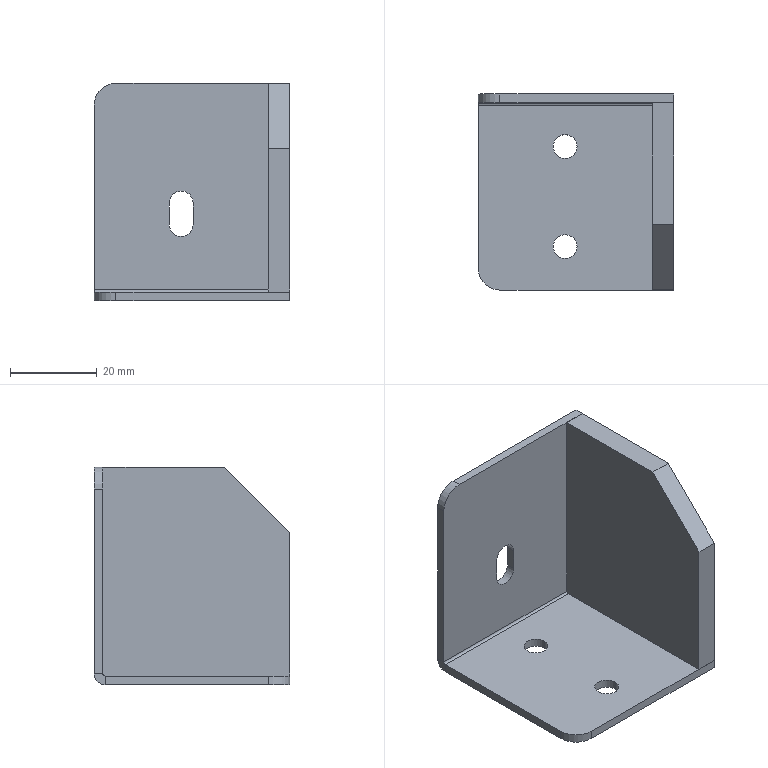Component | SolidWorks | 170423A4-ProfileSupportBlock-1 | 2 solids | 32 faces | box 45 x 45 x 50 mm | volume 17850 mm3 | plane 21 | cylinder 11 | commonest cylinder face diameters 5.5 x6 1 x2 10 x2 5 x1
STEP:
#1=COLOUR_RGB('',0.7922,0.8196,0.9333);
#2=FILL_AREA_STYLE_COLOUR('',#1);
#3=FILL_AREA_STYLE('',(#2));
#4=SURFACE_STYLE_FILL_AREA(#3);
#5=SURFACE_SIDE_STYLE('',(#4));
#6=SURFACE_STYLE_USAGE(.BOTH.,#5);
#7=PRESENTATION_STYLE_ASSIGNMENT((#6));
#8=CARTESIAN_POINT('',(3.248,-1.901,16.575));
#9=VERTEX_POINT('',#8);
#10=CARTESIAN_POINT('',(3.032,-1.901,16.575));
#11=VERTEX_POINT('',#10);
#12=CARTESIAN_POINT('',(3.14,-1.901,16.575));
#13=DIRECTION('',(0.,0.,1.));
#14=DIRECTION('',(-1.,0.,0.));
#15=AXIS2_PLACEMENT_3D('',#12,#13,#14);
#16=CIRCLE('',#15,0.1083);
#17=EDGE_CURVE('',#9,#11,#16,.T.);
#18=ORIENTED_EDGE('',*,*,#17,.F.);
#19=CARTESIAN_POINT('',(3.248,-1.901,16.654));
#20=VERTEX_POINT('',#19);
#21=CARTESIAN_POINT('',(3.248,-1.901,16.654));
#22=DIRECTION('',(0.,0.,1.));
#23=VECTOR('',#22,39.37);
#24=LINE('',#21,#23);
#25=EDGE_CURVE('',#9,#20,#24,.T.);
#26=ORIENTED_EDGE('',*,*,#25,.T.);
#27=CARTESIAN_POINT('',(3.032,-1.901,16.654));
#28=VERTEX_POINT('',#27);
#29=CARTESIAN_POINT('',(3.14,-1.901,16.654));
#30=DIRECTION('',(0.,0.,1.));
#31=DIRECTION('',(-1.,0.,0.));
#32=AXIS2_PLACEMENT_3D('',#29,#30,#31);
#33=CIRCLE('',#32,0.1083);
#34=EDGE_CURVE('',#20,#28,#33,.T.);
#35=ORIENTED_EDGE('',*,*,#34,.T.);
#36=CARTESIAN_POINT('',(3.032,-1.901,16.654));
#37=DIRECTION('',(0.,0.,1.));
#38=VECTOR('',#37,39.37);
#39=LINE('',#36,#38);
#40=EDGE_CURVE('',#11,#28,#39,.T.);
#41=ORIENTED_EDGE('',*,*,#40,.F.);
#42=EDGE_LOOP('',(#18,#26,#35,#41));
#43=FACE_OUTER_BOUND('',#42,.T.);
#44=CARTESIAN_POINT('',(3.14,-1.901,16.654));
#45=DIRECTION('',(0.,0.,1.));
#46=DIRECTION('',(-1.,0.,0.));
#47=AXIS2_PLACEMENT_3D('',#44,#45,#46);
#48=CYLINDRICAL_SURFACE('',#47,0.1083);
#49=ADVANCED_FACE('',(#43),#48,.F.);
#50=CARTESIAN_POINT('',(3.248,-2.807,16.575));
#51=VERTEX_POINT('',#50);
#52=CARTESIAN_POINT('',(3.032,-2.807,16.575));
#53=VERTEX_POINT('',#52);
#54=CARTESIAN_POINT('',(3.14,-2.807,16.575));
#55=DIRECTION('',(0.,0.,1.));
#56=DIRECTION('',(-1.,0.,0.));
#57=AXIS2_PLACEMENT_3D('',#54,#55,#56);
#58=CIRCLE('',#57,0.1083);
#59=EDGE_CURVE('',#51,#53,#58,.T.);
#60=ORIENTED_EDGE('',*,*,#59,.F.);
#61=CARTESIAN_POINT('',(3.248,-2.807,16.654));
#62=VERTEX_POINT('',#61);
#63=CARTESIAN_POINT('',(3.248,-2.807,16.654));
#64=DIRECTION('',(0.,0.,1.));
#65=VECTOR('',#64,39.37);
#66=LINE('',#63,#65);
#67=EDGE_CURVE('',#51,#62,#66,.T.);
#68=ORIENTED_EDGE('',*,*,#67,.T.);
#69=CARTESIAN_POINT('',(3.032,-2.807,16.654));
#70=VERTEX_POINT('',#69);
#71=CARTESIAN_POINT('',(3.14,-2.807,16.654));
#72=DIRECTION('',(0.,0.,1.));
#73=DIRECTION('',(-1.,0.,0.));
#74=AXIS2_PLACEMENT_3D('',#71,#72,#73);
#75=CIRCLE('',#74,0.1083);
#76=EDGE_CURVE('',#62,#70,#75,.T.);
#77=ORIENTED_EDGE('',*,*,#76,.T.);
#78=CARTESIAN_POINT('',(3.032,-2.807,16.654));
#79=DIRECTION('',(0.,0.,1.));
#80=VECTOR('',#79,39.37);
#81=LINE('',#78,#80);
#82=EDGE_CURVE('',#53,#70,#81,.T.);
#83=ORIENTED_EDGE('',*,*,#82,.F.);
#84=EDGE_LOOP('',(#60,#68,#77,#83));
#85=FACE_OUTER_BOUND('',#84,.T.);
#86=CARTESIAN_POINT('',(3.14,-2.807,16.654));
#87=DIRECTION('',(0.,0.,1.));
#88=DIRECTION('',(-1.,0.,0.));
#89=AXIS2_PLACEMENT_3D('',#86,#87,#88);
#90=CYLINDRICAL_SURFACE('',#89,0.1083);
#91=ADVANCED_FACE('',(#85),#90,.F.);
#92=CARTESIAN_POINT('',(2.353,-1.429,16.673));
#93=VERTEX_POINT('',#92);
#94=CARTESIAN_POINT('',(2.353,-1.507,16.673));
#95=VERTEX_POINT('',#94);
#96=CARTESIAN_POINT('',(2.353,-1.429,16.673));
#97=DIRECTION('',(0.,-1.,0.));
#98=VECTOR('',#97,39.37);
#99=LINE('',#96,#98);
#100=EDGE_CURVE('',#93,#95,#99,.T.);
#101=ORIENTED_EDGE('',*,*,#100,.F.);
#102=CARTESIAN_POINT('',(2.353,-1.527,16.575));
#103=VERTEX_POINT('',#102);
#104=CARTESIAN_POINT('',(2.353,-1.527,16.673));
#105=DIRECTION('',(-1.,-0.,0.));
#106=DIRECTION('',(0.,1.,0.));
#107=AXIS2_PLACEMENT_3D('',#104,#105,#106);
#108=CIRCLE('',#107,0.09843);
#109=EDGE_CURVE('',#93,#103,#108,.T.);
#110=ORIENTED_EDGE('',*,*,#109,.T.);
#111=CARTESIAN_POINT('',(2.353,-1.527,16.654));
#112=VERTEX_POINT('',#111);
#113=CARTESIAN_POINT('',(2.353,-1.527,16.654));
#114=DIRECTION('',(0.,0.,-1.));
#115=VECTOR('',#114,39.37);
#116=LINE('',#113,#115);
#117=EDGE_CURVE('',#112,#103,#116,.T.);
#118=ORIENTED_EDGE('',*,*,#117,.F.);
#119=CARTESIAN_POINT('',(2.353,-1.527,16.673));
#120=DIRECTION('',(-1.,-0.,0.));
#121=DIRECTION('',(0.,-1.,0.));
#122=AXIS2_PLACEMENT_3D('',#119,#120,#121);
#123=CIRCLE('',#122,0.01969);
#124=EDGE_CURVE('',#95,#112,#123,.T.);
#125=ORIENTED_EDGE('',*,*,#124,.F.);
#126=EDGE_LOOP('',(#101,#110,#118,#125));
#127=FACE_OUTER_BOUND('',#126,.T.);
#128=CARTESIAN_POINT('',(2.353,-1.429,16.673));
#129=DIRECTION('',(-1.,-0.,0.));
#130=DIRECTION('',(0.,-1.,0.));
#131=AXIS2_PLACEMENT_3D('',#128,#129,#130);
#132=PLANE('',#131);
#133=ADVANCED_FACE('',(#127),#132,.T.);
#134=CARTESIAN_POINT('',(2.353,-1.507,18.346));
#135=VERTEX_POINT('',#134);
#136=CARTESIAN_POINT('',(2.353,-1.507,16.575));
#137=DIRECTION('',(0.,0.,-1.));
#138=VECTOR('',#137,39.37);
#139=LINE('',#136,#138);
#140=EDGE_CURVE('',#135,#95,#139,.T.);
#141=ORIENTED_EDGE('',*,*,#140,.F.);
#142=CARTESIAN_POINT('',(2.353,-1.429,18.346));
#143=VERTEX_POINT('',#142);
#144=CARTESIAN_POINT('',(2.353,-1.527,18.346));
#145=DIRECTION('',(-0.,1.,0.));
#146=VECTOR('',#145,39.37);
#147=LINE('',#144,#146);
#148=EDGE_CURVE('',#135,#143,#147,.T.);
#149=ORIENTED_EDGE('',*,*,#148,.T.);
#150=CARTESIAN_POINT('',(2.353,-1.429,16.575));
#151=DIRECTION('',(0.,0.,-1.));
#152=VECTOR('',#151,39.37);
#153=LINE('',#150,#152);
#154=EDGE_CURVE('',#143,#93,#153,.T.);
#155=ORIENTED_EDGE('',*,*,#154,.T.);
#156=ORIENTED_EDGE('',*,*,#100,.T.);
#157=EDGE_LOOP('',(#141,#149,#155,#156));
#158=FACE_OUTER_BOUND('',#157,.T.);
#159=CARTESIAN_POINT('',(2.353,-1.527,16.654));
#160=DIRECTION('',(-1.,-0.,0.));
#161=DIRECTION('',(0.,-1.,0.));
#162=AXIS2_PLACEMENT_3D('',#159,#160,#161);
#163=PLANE('',#162);
#164=ADVANCED_FACE('',(#158),#163,.T.);
#165=CARTESIAN_POINT('',(4.124,-1.527,16.575));
#166=VERTEX_POINT('',#165);
#167=CARTESIAN_POINT('',(4.124,-1.527,16.654));
#168=VERTEX_POINT('',#167);
#169=CARTESIAN_POINT('',(4.124,-1.527,16.575));
#170=DIRECTION('',(0.,0.,1.));
#171=VECTOR('',#170,39.37);
#172=LINE('',#169,#171);
#173=EDGE_CURVE('',#166,#168,#172,.T.);
#174=ORIENTED_EDGE('',*,*,#173,.F.);
#175=CARTESIAN_POINT('',(4.124,-1.429,16.673));
#176=VERTEX_POINT('',#175);
#177=CARTESIAN_POINT('',(4.124,-1.527,16.673));
#178=DIRECTION('',(-1.,-0.,0.));
#179=DIRECTION('',(0.,1.,0.));
#180=AXIS2_PLACEMENT_3D('',#177,#178,#179);
#181=CIRCLE('',#180,0.09843);
#182=EDGE_CURVE('',#176,#166,#181,.T.);
#183=ORIENTED_EDGE('',*,*,#182,.F.);
#184=CARTESIAN_POINT('',(4.124,-1.507,16.673));
#185=VERTEX_POINT('',#184);
#186=CARTESIAN_POINT('',(4.124,-1.507,16.673));
#187=DIRECTION('',(-0.,1.,0.));
#188=VECTOR('',#187,39.37);
#189=LINE('',#186,#188);
#190=EDGE_CURVE('',#185,#176,#189,.T.);
#191=ORIENTED_EDGE('',*,*,#190,.F.);
#192=CARTESIAN_POINT('',(4.124,-1.527,16.673));
#193=DIRECTION('',(-1.,-0.,0.));
#194=DIRECTION('',(0.,-1.,0.));
#195=AXIS2_PLACEMENT_3D('',#192,#193,#194);
#196=CIRCLE('',#195,0.01969);
#197=EDGE_CURVE('',#185,#168,#196,.T.);
#198=ORIENTED_EDGE('',*,*,#197,.T.);
#199=EDGE_LOOP('',(#174,#183,#191,#198));
#200=FACE_OUTER_BOUND('',#199,.T.);
#201=CARTESIAN_POINT('',(4.124,-1.527,16.575));
#202=DIRECTION('',(1.,0.,0.));
#203=DIRECTION('',(-0.,1.,0.));
#204=AXIS2_PLACEMENT_3D('',#201,#202,#203);
#205=PLANE('',#204);
#206=ADVANCED_FACE('',(#200),#205,.T.);
#207=CARTESIAN_POINT('',(4.124,-3.2,16.575));
#208=VERTEX_POINT('',#207);
#209=CARTESIAN_POINT('',(4.124,-1.429,16.575));
#210=DIRECTION('',(0.,-1.,0.));
#211=VECTOR('',#210,39.37);
#212=LINE('',#209,#211);
#213=EDGE_CURVE('',#166,#208,#212,.T.);
#214=ORIENTED_EDGE('',*,*,#213,.F.);
#215=ORIENTED_EDGE('',*,*,#173,.T.);
#216=CARTESIAN_POINT('',(4.124,-3.2,16.654));
#217=VERTEX_POINT('',#216);
#218=CARTESIAN_POINT('',(4.124,-1.429,16.654));
#219=DIRECTION('',(0.,-1.,0.));
#220=VECTOR('',#219,39.37);
#221=LINE('',#218,#220);
#222=EDGE_CURVE('',#168,#217,#221,.T.);
#223=ORIENTED_EDGE('',*,*,#222,.T.);
#224=CARTESIAN_POINT('',(4.124,-3.2,16.654));
#225=DIRECTION('',(0.,0.,-1.));
#226=VECTOR('',#225,39.37);
#227=LINE('',#224,#226);
#228=EDGE_CURVE('',#217,#208,#227,.T.);
#229=ORIENTED_EDGE('',*,*,#228,.T.);
#230=EDGE_LOOP('',(#214,#215,#223,#229));
#231=FACE_OUTER_BOUND('',#230,.T.);
#232=CARTESIAN_POINT('',(4.124,-1.507,16.673));
#233=DIRECTION('',(1.,0.,0.));
#234=DIRECTION('',(-0.,1.,0.));
#235=AXIS2_PLACEMENT_3D('',#232,#233,#234);
#236=PLANE('',#235);
#237=ADVANCED_FACE('',(#231),#236,.T.);
#238=CARTESIAN_POINT('',(3.14,-1.901,16.575));
#239=DIRECTION('',(0.,0.,1.));
#240=DIRECTION('',(-1.,0.,0.));
#241=AXIS2_PLACEMENT_3D('',#238,#239,#240);
#242=CIRCLE('',#241,0.1083);
#243=EDGE_CURVE('',#11,#9,#242,.T.);
#244=ORIENTED_EDGE('',*,*,#243,.T.);
#245=ORIENTED_EDGE('',*,*,#17,.T.);
#246=EDGE_LOOP('',(#244,#245));
#247=FACE_BOUND('',#246,.T.);
#248=CARTESIAN_POINT('',(3.14,-2.807,16.575));
#249=DIRECTION('',(0.,0.,1.));
#250=DIRECTION('',(-1.,0.,0.));
#251=AXIS2_PLACEMENT_3D('',#248,#249,#250);
#252=CIRCLE('',#251,0.1083);
#253=EDGE_CURVE('',#53,#51,#252,.T.);
#254=ORIENTED_EDGE('',*,*,#253,.T.);
#255=ORIENTED_EDGE('',*,*,#59,.T.);
#256=EDGE_LOOP('',(#254,#255));
#257=FACE_BOUND('',#256,.T.);
#258=CARTESIAN_POINT('',(2.549,-3.2,16.575));
#259=VERTEX_POINT('',#258);
#260=CARTESIAN_POINT('',(2.353,-3.2,16.575));
#261=DIRECTION('',(1.,0.,0.));
#262=VECTOR('',#261,39.37);
#263=LINE('',#260,#262);
#264=EDGE_CURVE('',#259,#208,#263,.T.);
#265=ORIENTED_EDGE('',*,*,#264,.F.);
#266=CARTESIAN_POINT('',(2.353,-3.003,16.575));
#267=VERTEX_POINT('',#266);
#268=CARTESIAN_POINT('',(2.549,-3.003,16.575));
#269=DIRECTION('',(0.,0.,-1.));
#270=DIRECTION('',(-1.,-0.,0.));
#271=AXIS2_PLACEMENT_3D('',#268,#269,#270);
#272=CIRCLE('',#271,0.1969);
#273=EDGE_CURVE('',#259,#267,#272,.T.);
#274=ORIENTED_EDGE('',*,*,#273,.T.);
#275=CARTESIAN_POINT('',(2.353,-1.429,16.575));
#276=DIRECTION('',(0.,-1.,0.));
#277=VECTOR('',#276,39.37);
#278=LINE('',#275,#277);
#279=EDGE_CURVE('',#103,#267,#278,.T.);
#280=ORIENTED_EDGE('',*,*,#279,.F.);
#281=CARTESIAN_POINT('',(2.353,-1.527,16.575));
#282=DIRECTION('',(1.,0.,0.));
#283=VECTOR('',#282,39.37);
#284=LINE('',#281,#283);
#285=EDGE_CURVE('',#103,#166,#284,.T.);
#286=ORIENTED_EDGE('',*,*,#285,.T.);
#287=ORIENTED_EDGE('',*,*,#213,.T.);
#288=EDGE_LOOP('',(#265,#274,#280,#286,#287));
#289=FACE_OUTER_BOUND('',#288,.T.);
#290=CARTESIAN_POINT('',(2.353,-1.429,16.575));
#291=DIRECTION('',(0.,0.,1.));
#292=DIRECTION('',(-1.,-0.,0.));
#293=AXIS2_PLACEMENT_3D('',#290,#291,#292);
#294=PLANE('',#293);
#295=ADVANCED_FACE('',(#247,#257,#289),#294,.F.);
#296=CARTESIAN_POINT('',(2.549,-3.2,16.654));
#297=VERTEX_POINT('',#296);
#298=CARTESIAN_POINT('',(2.353,-3.2,16.654));
#299=DIRECTION('',(1.,0.,0.));
#300=VECTOR('',#299,39.37);
#301=LINE('',#298,#300);
#302=EDGE_CURVE('',#297,#217,#301,.T.);
#303=ORIENTED_EDGE('',*,*,#302,.F.);
#304=CARTESIAN_POINT('',(2.549,-3.2,16.654));
#305=DIRECTION('',(0.,0.,-1.));
#306=VECTOR('',#305,39.37);
#307=LINE('',#304,#306);
#308=EDGE_CURVE('',#297,#259,#307,.T.);
#309=ORIENTED_EDGE('',*,*,#308,.T.);
#310=ORIENTED_EDGE('',*,*,#264,.T.);
#311=ORIENTED_EDGE('',*,*,#228,.F.);
#312=EDGE_LOOP('',(#303,#309,#310,#311));
#313=FACE_OUTER_BOUND('',#312,.T.);
#314=CARTESIAN_POINT('',(2.353,-3.2,16.654));
#315=DIRECTION('',(0.,-1.,0.));
#316=DIRECTION('',(1.,0.,0.));
#317=AXIS2_PLACEMENT_3D('',#314,#315,#316);
#318=PLANE('',#317);
#319=ADVANCED_FACE('',(#313),#318,.T.);
#320=CARTESIAN_POINT('',(3.14,-1.901,16.654));
#321=DIRECTION('',(0.,0.,1.));
#322=DIRECTION('',(-1.,0.,0.));
#323=AXIS2_PLACEMENT_3D('',#320,#321,#322);
#324=CIRCLE('',#323,0.1083);
#325=EDGE_CURVE('',#28,#20,#324,.T.);
#326=ORIENTED_EDGE('',*,*,#325,.F.);
#327=ORIENTED_EDGE('',*,*,#34,.F.);
#328=EDGE_LOOP('',(#326,#327));
#329=FACE_BOUND('',#328,.T.);
#330=CARTESIAN_POINT('',(3.14,-2.807,16.654));
#331=DIRECTION('',(0.,0.,1.));
#332=DIRECTION('',(-1.,0.,0.));
#333=AXIS2_PLACEMENT_3D('',#330,#331,#332);
#334=CIRCLE('',#333,0.1083);
#335=EDGE_CURVE('',#70,#62,#334,.T.);
#336=ORIENTED_EDGE('',*,*,#335,.F.);
#337=ORIENTED_EDGE('',*,*,#76,.F.);
#338=EDGE_LOOP('',(#336,#337));
#339=FACE_BOUND('',#338,.T.);
#340=CARTESIAN_POINT('',(2.353,-3.003,16.654));
#341=VERTEX_POINT('',#340);
#342=CARTESIAN_POINT('',(2.353,-1.429,16.654));
#343=DIRECTION('',(0.,-1.,0.));
#344=VECTOR('',#343,39.37);
#345=LINE('',#342,#344);
#346=EDGE_CURVE('',#112,#341,#345,.T.);
#347=ORIENTED_EDGE('',*,*,#346,.T.);
#348=CARTESIAN_POINT('',(2.549,-3.003,16.654));
#349=DIRECTION('',(0.,0.,1.));
#350=DIRECTION('',(-1.,0.,0.));
#351=AXIS2_PLACEMENT_3D('',#348,#349,#350);
#352=CIRCLE('',#351,0.1969);
#353=EDGE_CURVE('',#341,#297,#352,.T.);
#354=ORIENTED_EDGE('',*,*,#353,.T.);
#355=ORIENTED_EDGE('',*,*,#302,.T.);
#356=ORIENTED_EDGE('',*,*,#222,.F.);
#357=CARTESIAN_POINT('',(2.353,-1.527,16.654));
#358=DIRECTION('',(1.,0.,0.));
#359=VECTOR('',#358,39.37);
#360=LINE('',#357,#359);
#361=EDGE_CURVE('',#112,#168,#360,.T.);
#362=ORIENTED_EDGE('',*,*,#361,.F.);
#363=EDGE_LOOP('',(#347,#354,#355,#356,#362));
#364=FACE_OUTER_BOUND('',#363,.T.);
#365=CARTESIAN_POINT('',(2.353,-1.429,16.654));
#366=DIRECTION('',(0.,0.,1.));
#367=DIRECTION('',(-1.,-0.,0.));
#368=AXIS2_PLACEMENT_3D('',#365,#366,#367);
#369=PLANE('',#368);
#370=ADVANCED_FACE('',(#329,#339,#364),#369,.T.);
#371=ORIENTED_EDGE('',*,*,#197,.F.);
#372=CARTESIAN_POINT('',(2.353,-1.507,16.673));
#373=DIRECTION('',(1.,0.,0.));
#374=VECTOR('',#373,39.37);
#375=LINE('',#372,#374);
#376=EDGE_CURVE('',#95,#185,#375,.T.);
#377=ORIENTED_EDGE('',*,*,#376,.F.);
#378=ORIENTED_EDGE('',*,*,#124,.T.);
#379=ORIENTED_EDGE('',*,*,#361,.T.);
#380=EDGE_LOOP('',(#371,#377,#378,#379));
#381=FACE_OUTER_BOUND('',#380,.T.);
#382=CARTESIAN_POINT('',(2.353,-1.527,16.673));
#383=DIRECTION('',(1.,0.,0.));
#384=DIRECTION('',(0.,1.,0.));
#385=AXIS2_PLACEMENT_3D('',#382,#383,#384);
#386=CYLINDRICAL_SURFACE('',#385,0.01969);
#387=ADVANCED_FACE('',(#381),#386,.F.);
#388=CARTESIAN_POINT('',(3.032,-1.507,17.264));
#389=VERTEX_POINT('',#388);
#390=CARTESIAN_POINT('',(3.248,-1.507,17.264));
#391=VERTEX_POINT('',#390);
#392=CARTESIAN_POINT('',(3.14,-1.507,17.264));
#393=DIRECTION('',(0.,-1.,0.));
#394=DIRECTION('',(1.,0.,0.));
#395=AXIS2_PLACEMENT_3D('',#392,#393,#394);
#396=CIRCLE('',#395,0.1083);
#397=EDGE_CURVE('',#389,#391,#396,.T.);
#398=ORIENTED_EDGE('',*,*,#397,.F.);
#399=CARTESIAN_POINT('',(3.032,-1.507,17.461));
#400=VERTEX_POINT('',#399);
#401=CARTESIAN_POINT('',(3.032,-1.507,17.264));
#402=DIRECTION('',(0.,0.,-1.));
#403=VECTOR('',#402,39.37);
#404=LINE('',#401,#403);
#405=EDGE_CURVE('',#400,#389,#404,.T.);
#406=ORIENTED_EDGE('',*,*,#405,.F.);
#407=CARTESIAN_POINT('',(3.248,-1.507,17.461));
#408=VERTEX_POINT('',#407);
#409=CARTESIAN_POINT('',(3.14,-1.507,17.461));
#410=DIRECTION('',(0.,-1.,0.));
#411=DIRECTION('',(1.,0.,0.));
#412=AXIS2_PLACEMENT_3D('',#409,#410,#411);
#413=CIRCLE('',#412,0.1083);
#414=EDGE_CURVE('',#408,#400,#413,.T.);
#415=ORIENTED_EDGE('',*,*,#414,.F.);
#416=CARTESIAN_POINT('',(3.248,-1.507,17.264));
#417=DIRECTION('',(0.,0.,1.));
#418=VECTOR('',#417,39.37);
#419=LINE('',#416,#418);
#420=EDGE_CURVE('',#391,#408,#419,.T.);
#421=ORIENTED_EDGE('',*,*,#420,.F.);
#422=EDGE_LOOP('',(#398,#406,#415,#421));
#423=FACE_BOUND('',#422,.T.);
#424=CARTESIAN_POINT('',(2.549,-1.507,18.543));
#425=VERTEX_POINT('',#424);
#426=CARTESIAN_POINT('',(4.124,-1.507,18.543));
#427=VERTEX_POINT('',#426);
#428=CARTESIAN_POINT('',(2.353,-1.507,18.543));
#429=DIRECTION('',(1.,0.,0.));
#430=VECTOR('',#429,39.37);
#431=LINE('',#428,#430);
#432=EDGE_CURVE('',#425,#427,#431,.T.);
#433=ORIENTED_EDGE('',*,*,#432,.F.);
#434=CARTESIAN_POINT('',(2.549,-1.507,18.346));
#435=DIRECTION('',(0.,-1.,0.));
#436=DIRECTION('',(1.,0.,0.));
#437=AXIS2_PLACEMENT_3D('',#434,#435,#436);
#438=CIRCLE('',#437,0.1969);
#439=EDGE_CURVE('',#425,#135,#438,.T.);
#440=ORIENTED_EDGE('',*,*,#439,.T.);
#441=ORIENTED_EDGE('',*,*,#140,.T.);
#442=ORIENTED_EDGE('',*,*,#376,.T.);
#443=CARTESIAN_POINT('',(4.124,-1.507,16.575));
#444=DIRECTION('',(0.,0.,-1.));
#445=VECTOR('',#444,39.37);
#446=LINE('',#443,#445);
#447=EDGE_CURVE('',#427,#185,#446,.T.);
#448=ORIENTED_EDGE('',*,*,#447,.F.);
#449=EDGE_LOOP('',(#433,#440,#441,#442,#448));
#450=FACE_OUTER_BOUND('',#449,.T.);
#451=CARTESIAN_POINT('',(2.353,-1.507,16.575));
#452=DIRECTION('',(0.,-1.,0.));
#453=DIRECTION('',(1.,0.,0.));
#454=AXIS2_PLACEMENT_3D('',#451,#452,#453);
#455=PLANE('',#454);
#456=ADVANCED_FACE('',(#423,#450),#455,.T.);
#457=CARTESIAN_POINT('',(2.549,-1.429,18.543));
#458=VERTEX_POINT('',#457);
#459=CARTESIAN_POINT('',(4.124,-1.429,18.543));
#460=VERTEX_POINT('',#459);
#461=CARTESIAN_POINT('',(2.353,-1.429,18.543));
#462=DIRECTION('',(1.,0.,0.));
#463=VECTOR('',#462,39.37);
#464=LINE('',#461,#463);
#465=EDGE_CURVE('',#458,#460,#464,.T.);
#466=ORIENTED_EDGE('',*,*,#465,.F.);
#467=CARTESIAN_POINT('',(2.549,-1.429,18.543));
#468=DIRECTION('',(0.,-1.,0.));
#469=VECTOR('',#468,39.37);
#470=LINE('',#467,#469);
#471=EDGE_CURVE('',#458,#425,#470,.T.);
#472=ORIENTED_EDGE('',*,*,#471,.T.);
#473=ORIENTED_EDGE('',*,*,#432,.T.);
#474=CARTESIAN_POINT('',(4.124,-1.429,18.543));
#475=DIRECTION('',(0.,-1.,0.));
#476=VECTOR('',#475,39.37);
#477=LINE('',#474,#476);
#478=EDGE_CURVE('',#460,#427,#477,.T.);
#479=ORIENTED_EDGE('',*,*,#478,.F.);
#480=EDGE_LOOP('',(#466,#472,#473,#479));
#481=FACE_OUTER_BOUND('',#480,.T.);
#482=CARTESIAN_POINT('',(2.353,-1.429,18.543));
#483=DIRECTION('',(0.,0.,1.));
#484=DIRECTION('',(-1.,-0.,0.));
#485=AXIS2_PLACEMENT_3D('',#482,#483,#484);
#486=PLANE('',#485);
#487=ADVANCED_FACE('',(#481),#486,.T.);
#488=CARTESIAN_POINT('',(3.032,-1.429,17.461));
#489=VERTEX_POINT('',#488);
#490=CARTESIAN_POINT('',(3.032,-1.429,17.264));
#491=VERTEX_POINT('',#490);
#492=CARTESIAN_POINT('',(3.032,-1.429,17.264));
#493=DIRECTION('',(0.,0.,-1.));
#494=VECTOR('',#493,39.37);
#495=LINE('',#492,#494);
#496=EDGE_CURVE('',#489,#491,#495,.T.);
#497=ORIENTED_EDGE('',*,*,#496,.T.);
#498=CARTESIAN_POINT('',(3.248,-1.429,17.264));
#499=VERTEX_POINT('',#498);
#500=CARTESIAN_POINT('',(3.14,-1.429,17.264));
#501=DIRECTION('',(0.,-1.,0.));
#502=DIRECTION('',(1.,0.,0.));
#503=AXIS2_PLACEMENT_3D('',#500,#501,#502);
#504=CIRCLE('',#503,0.1083);
#505=EDGE_CURVE('',#491,#499,#504,.T.);
#506=ORIENTED_EDGE('',*,*,#505,.T.);
#507=CARTESIAN_POINT('',(3.248,-1.429,17.461));
#508=VERTEX_POINT('',#507);
#509=CARTESIAN_POINT('',(3.248,-1.429,17.264));
#510=DIRECTION('',(0.,0.,1.));
#511=VECTOR('',#510,39.37);
#512=LINE('',#509,#511);
#513=EDGE_CURVE('',#499,#508,#512,.T.);
#514=ORIENTED_EDGE('',*,*,#513,.T.);
#515=CARTESIAN_POINT('',(3.14,-1.429,17.461));
#516=DIRECTION('',(0.,-1.,0.));
#517=DIRECTION('',(1.,0.,0.));
#518=AXIS2_PLACEMENT_3D('',#515,#516,#517);
#519=CIRCLE('',#518,0.1083);
#520=EDGE_CURVE('',#508,#489,#519,.T.);
#521=ORIENTED_EDGE('',*,*,#520,.T.);
#522=EDGE_LOOP('',(#497,#506,#514,#521));
#523=FACE_BOUND('',#522,.T.);
#524=ORIENTED_EDGE('',*,*,#154,.F.);
#525=CARTESIAN_POINT('',(2.549,-1.429,18.346));
#526=DIRECTION('',(-0.,1.,0.));
#527=DIRECTION('',(1.,0.,0.));
#528=AXIS2_PLACEMENT_3D('',#525,#526,#527);
#529=CIRCLE('',#528,0.1969);
#530=EDGE_CURVE('',#143,#458,#529,.T.);
#531=ORIENTED_EDGE('',*,*,#530,.T.);
#532=ORIENTED_EDGE('',*,*,#465,.T.);
#533=CARTESIAN_POINT('',(4.124,-1.429,16.575));
#534=DIRECTION('',(0.,0.,-1.));
#535=VECTOR('',#534,39.37);
#536=LINE('',#533,#535);
#537=EDGE_CURVE('',#460,#176,#536,.T.);
#538=ORIENTED_EDGE('',*,*,#537,.T.);
#539=CARTESIAN_POINT('',(2.353,-1.429,16.673));
#540=DIRECTION('',(1.,0.,0.));
#541=VECTOR('',#540,39.37);
#542=LINE('',#539,#541);
#543=EDGE_CURVE('',#93,#176,#542,.T.);
#544=ORIENTED_EDGE('',*,*,#543,.F.);
#545=EDGE_LOOP('',(#524,#531,#532,#538,#544));
#546=FACE_OUTER_BOUND('',#545,.T.);
#547=CARTESIAN_POINT('',(2.353,-1.429,16.575));
#548=DIRECTION('',(0.,-1.,0.));
#549=DIRECTION('',(1.,0.,0.));
#550=AXIS2_PLACEMENT_3D('',#547,#548,#549);
#551=PLANE('',#550);
#552=ADVANCED_FACE('',(#523,#546),#551,.F.);
#553=ORIENTED_EDGE('',*,*,#182,.T.);
#554=ORIENTED_EDGE('',*,*,#285,.F.);
#555=ORIENTED_EDGE('',*,*,#109,.F.);
#556=ORIENTED_EDGE('',*,*,#543,.T.);
#557=EDGE_LOOP('',(#553,#554,#555,#556));
#558=FACE_OUTER_BOUND('',#557,.T.);
#559=CARTESIAN_POINT('',(2.353,-1.527,16.673));
#560=DIRECTION('',(1.,0.,0.));
#561=DIRECTION('',(0.,1.,0.));
#562=AXIS2_PLACEMENT_3D('',#559,#560,#561);
#563=CYLINDRICAL_SURFACE('',#562,0.09843);
#564=ADVANCED_FACE('',(#558),#563,.T.);
#565=ORIENTED_EDGE('',*,*,#279,.T.);
#566=CARTESIAN_POINT('',(2.353,-3.003,16.673));
#567=DIRECTION('',(0.,0.,1.));
#568=VECTOR('',#567,39.37);
#569=LINE('',#566,#568);
#570=EDGE_CURVE('',#267,#341,#569,.T.);
#571=ORIENTED_EDGE('',*,*,#570,.T.);
#572=ORIENTED_EDGE('',*,*,#346,.F.);
#573=ORIENTED_EDGE('',*,*,#117,.T.);
#574=EDGE_LOOP('',(#565,#571,#572,#573));
#575=FACE_OUTER_BOUND('',#574,.T.);
#576=CARTESIAN_POINT('',(2.353,-1.527,16.673));
#577=DIRECTION('',(-1.,-0.,0.));
#578=DIRECTION('',(0.,-1.,0.));
#579=AXIS2_PLACEMENT_3D('',#576,#577,#578);
#580=PLANE('',#579);
#581=ADVANCED_FACE('',(#575),#580,.T.);
#582=ORIENTED_EDGE('',*,*,#447,.T.);
#583=ORIENTED_EDGE('',*,*,#190,.T.);
#584=ORIENTED_EDGE('',*,*,#537,.F.);
#585=ORIENTED_EDGE('',*,*,#478,.T.);
#586=EDGE_LOOP('',(#582,#583,#584,#585));
#587=FACE_OUTER_BOUND('',#586,.T.);
#588=CARTESIAN_POINT('',(4.124,-1.527,16.673));
#589=DIRECTION('',(-1.,-0.,0.));
#590=DIRECTION('',(0.,-1.,0.));
#591=AXIS2_PLACEMENT_3D('',#588,#589,#590);
#592=PLANE('',#591);
#593=ADVANCED_FACE('',(#587),#592,.F.);
#594=ORIENTED_EDGE('',*,*,#397,.T.);
#595=CARTESIAN_POINT('',(3.248,-1.429,17.264));
#596=DIRECTION('',(0.,-1.,0.));
#597=VECTOR('',#596,39.37);
#598=LINE('',#595,#597);
#599=EDGE_CURVE('',#499,#391,#598,.T.);
#600=ORIENTED_EDGE('',*,*,#599,.F.);
#601=ORIENTED_EDGE('',*,*,#505,.F.);
#602=CARTESIAN_POINT('',(3.032,-1.429,17.264));
#603=DIRECTION('',(0.,-1.,0.));
#604=VECTOR('',#603,39.37);
#605=LINE('',#602,#604);
#606=EDGE_CURVE('',#491,#389,#605,.T.);
#607=ORIENTED_EDGE('',*,*,#606,.T.);
#608=EDGE_LOOP('',(#594,#600,#601,#607));
#609=FACE_OUTER_BOUND('',#608,.T.);
#610=CARTESIAN_POINT('',(3.14,-1.429,17.264));
#611=DIRECTION('',(0.,-1.,0.));
#612=DIRECTION('',(1.,0.,0.));
#613=AXIS2_PLACEMENT_3D('',#610,#611,#612);
#614=CYLINDRICAL_SURFACE('',#613,0.1083);
#615=ADVANCED_FACE('',(#609),#614,.F.);
#616=ORIENTED_EDGE('',*,*,#405,.T.);
#617=ORIENTED_EDGE('',*,*,#606,.F.);
#618=ORIENTED_EDGE('',*,*,#496,.F.);
#619=CARTESIAN_POINT('',(3.032,-1.429,17.461));
#620=DIRECTION('',(0.,-1.,0.));
#621=VECTOR('',#620,39.37);
#622=LINE('',#619,#621);
#623=EDGE_CURVE('',#489,#400,#622,.T.);
#624=ORIENTED_EDGE('',*,*,#623,.T.);
#625=EDGE_LOOP('',(#616,#617,#618,#624));
#626=FACE_OUTER_BOUND('',#625,.T.);
#627=CARTESIAN_POINT('',(3.032,-1.429,17.264));
#628=DIRECTION('',(-1.,-0.,0.));
#629=DIRECTION('',(0.,-1.,0.));
#630=AXIS2_PLACEMENT_3D('',#627,#628,#629);
#631=PLANE('',#630);
#632=ADVANCED_FACE('',(#626),#631,.F.);
#633=ORIENTED_EDGE('',*,*,#414,.T.);
#634=ORIENTED_EDGE('',*,*,#623,.F.);
#635=ORIENTED_EDGE('',*,*,#520,.F.);
#636=CARTESIAN_POINT('',(3.248,-1.429,17.461));
#637=DIRECTION('',(0.,-1.,0.));
#638=VECTOR('',#637,39.37);
#639=LINE('',#636,#638);
#640=EDGE_CURVE('',#508,#408,#639,.T.);
#641=ORIENTED_EDGE('',*,*,#640,.T.);
#642=EDGE_LOOP('',(#633,#634,#635,#641));
#643=FACE_OUTER_BOUND('',#642,.T.);
#644=CARTESIAN_POINT('',(3.14,-1.429,17.461));
#645=DIRECTION('',(0.,-1.,0.));
#646=DIRECTION('',(1.,0.,0.));
#647=AXIS2_PLACEMENT_3D('',#644,#645,#646);
#648=CYLINDRICAL_SURFACE('',#647,0.1083);
#649=ADVANCED_FACE('',(#643),#648,.F.);
#650=ORIENTED_EDGE('',*,*,#420,.T.);
#651=ORIENTED_EDGE('',*,*,#640,.F.);
#652=ORIENTED_EDGE('',*,*,#513,.F.);
#653=ORIENTED_EDGE('',*,*,#599,.T.);
#654=EDGE_LOOP('',(#650,#651,#652,#653));
#655=FACE_OUTER_BOUND('',#654,.T.);
#656=CARTESIAN_POINT('',(3.248,-1.429,17.264));
#657=DIRECTION('',(1.,0.,0.));
#658=DIRECTION('',(-0.,1.,0.));
#659=AXIS2_PLACEMENT_3D('',#656,#657,#658);
#660=PLANE('',#659);
#661=ADVANCED_FACE('',(#655),#660,.F.);
#662=ORIENTED_EDGE('',*,*,#353,.F.);
#663=ORIENTED_EDGE('',*,*,#570,.F.);
#664=ORIENTED_EDGE('',*,*,#273,.F.);
#665=ORIENTED_EDGE('',*,*,#308,.F.);
#666=EDGE_LOOP('',(#662,#663,#664,#665));
#667=FACE_OUTER_BOUND('',#666,.T.);
#668=CARTESIAN_POINT('',(2.549,-3.003,16.654));
#669=DIRECTION('',(0.,0.,-1.));
#670=DIRECTION('',(1.,0.,0.));
#671=AXIS2_PLACEMENT_3D('',#668,#669,#670);
#672=CYLINDRICAL_SURFACE('',#671,0.1969);
#673=ADVANCED_FACE('',(#667),#672,.T.);
#674=ORIENTED_EDGE('',*,*,#530,.F.);
#675=ORIENTED_EDGE('',*,*,#148,.F.);
#676=ORIENTED_EDGE('',*,*,#439,.F.);
#677=ORIENTED_EDGE('',*,*,#471,.F.);
#678=EDGE_LOOP('',(#674,#675,#676,#677));
#679=FACE_OUTER_BOUND('',#678,.T.);
#680=CARTESIAN_POINT('',(2.549,-1.429,18.346));
#681=DIRECTION('',(0.,-1.,0.));
#682=DIRECTION('',(1.,0.,0.));
#683=AXIS2_PLACEMENT_3D('',#680,#681,#682);
#684=CYLINDRICAL_SURFACE('',#683,0.1969);
#685=ADVANCED_FACE('',(#679),#684,.T.);
#686=ORIENTED_EDGE('',*,*,#67,.F.);
#687=ORIENTED_EDGE('',*,*,#253,.F.);
#688=ORIENTED_EDGE('',*,*,#82,.T.);
#689=ORIENTED_EDGE('',*,*,#335,.T.);
#690=EDGE_LOOP('',(#686,#687,#688,#689));
#691=FACE_OUTER_BOUND('',#690,.T.);
#692=CARTESIAN_POINT('',(3.14,-2.807,16.654));
#693=DIRECTION('',(0.,0.,1.));
#694=DIRECTION('',(-1.,0.,0.));
#695=AXIS2_PLACEMENT_3D('',#692,#693,#694);
#696=CYLINDRICAL_SURFACE('',#695,0.1083);
#697=ADVANCED_FACE('',(#691),#696,.F.);
#698=ORIENTED_EDGE('',*,*,#25,.F.);
#699=ORIENTED_EDGE('',*,*,#243,.F.);
#700=ORIENTED_EDGE('',*,*,#40,.T.);
#701=ORIENTED_EDGE('',*,*,#325,.T.);
#702=EDGE_LOOP('',(#698,#699,#700,#701));
#703=FACE_OUTER_BOUND('',#702,.T.);
#704=CARTESIAN_POINT('',(3.14,-1.901,16.654));
#705=DIRECTION('',(0.,0.,1.));
#706=DIRECTION('',(-1.,0.,0.));
#707=AXIS2_PLACEMENT_3D('',#704,#705,#706);
#708=CYLINDRICAL_SURFACE('',#707,0.1083);
#709=ADVANCED_FACE('',(#703),#708,.F.);
#710=CLOSED_SHELL('',(#49,#91,#133,#164,#206,#237,#295,#319,#370,#387,#456,#487,#552,#564,#581,#593,#615,#632,#649,#661,#673,#685,#697,#709));
#711=MANIFOLD_SOLID_BREP('',#710);
#712=STYLED_ITEM('',(#7),#711);
#713=(LENGTH_UNIT()NAMED_UNIT(*)SI_UNIT($,.METRE.));
#714=LENGTH_MEASURE_WITH_UNIT(LENGTH_MEASURE(0.0254),#713);
#715=DIMENSIONAL_EXPONENTS(1.,0.,0.,0.,0.,0.,0.);
#716=(CONVERSION_BASED_UNIT('',#714)LENGTH_UNIT()NAMED_UNIT(#715));
#717=UNCERTAINTY_MEASURE_WITH_UNIT(LENGTH_MEASURE(0.00001),#716,'','');
#718=(NAMED_UNIT(*)PLANE_ANGLE_UNIT()SI_UNIT($,.RADIAN.));
#719=(NAMED_UNIT(*)SI_UNIT($,.STERADIAN.)SOLID_ANGLE_UNIT());
#720=(GEOMETRIC_REPRESENTATION_CONTEXT(3)GLOBAL_UNCERTAINTY_ASSIGNED_CONTEXT((#717))GLOBAL_UNIT_ASSIGNED_CONTEXT((#716,#718,#719))REPRESENTATION_CONTEXT('',''));
#721=MECHANICAL_DESIGN_GEOMETRIC_PRESENTATION_REPRESENTATION('',(#712),#720);
#722=COLOUR_RGB('',0.7922,0.8196,0.9333);
#723=FILL_AREA_STYLE_COLOUR('',#722);
#724=FILL_AREA_STYLE('',(#723));
#725=SURFACE_STYLE_FILL_AREA(#724);
#726=SURFACE_SIDE_STYLE('',(#725));
#727=SURFACE_STYLE_USAGE(.BOTH.,#726);
#728=PRESENTATION_STYLE_ASSIGNMENT((#727));
#729=CARTESIAN_POINT('',(4.124,-1.527,16.654));
#730=VERTEX_POINT('',#729);
#731=CARTESIAN_POINT('',(4.124,-1.507,16.673));
#732=VERTEX_POINT('',#731);
#733=CARTESIAN_POINT('',(4.124,-1.527,16.673));
#734=DIRECTION('',(1.,0.,0.));
#735=DIRECTION('',(0.,1.,0.));
#736=AXIS2_PLACEMENT_3D('',#733,#734,#735);
#737=CIRCLE('',#736,0.01969);
#738=EDGE_CURVE('',#730,#732,#737,.T.);
#739=ORIENTED_EDGE('',*,*,#738,.F.);
#740=CARTESIAN_POINT('',(3.927,-1.527,16.654));
#741=VERTEX_POINT('',#740);
#742=CARTESIAN_POINT('',(3.927,-1.527,16.654));
#743=DIRECTION('',(1.,0.,0.));
#744=VECTOR('',#743,39.37);
#745=LINE('',#742,#744);
#746=EDGE_CURVE('',#741,#730,#745,.T.);
#747=ORIENTED_EDGE('',*,*,#746,.F.);
#748=CARTESIAN_POINT('',(3.927,-1.507,16.673));
#749=VERTEX_POINT('',#748);
#750=CARTESIAN_POINT('',(3.927,-1.527,16.673));
#751=DIRECTION('',(1.,0.,0.));
#752=DIRECTION('',(0.,1.,0.));
#753=AXIS2_PLACEMENT_3D('',#750,#751,#752);
#754=CIRCLE('',#753,0.01969);
#755=EDGE_CURVE('',#741,#749,#754,.T.);
#756=ORIENTED_EDGE('',*,*,#755,.T.);
#757=CARTESIAN_POINT('',(3.927,-1.507,16.673));
#758=DIRECTION('',(1.,0.,0.));
#759=VECTOR('',#758,39.37);
#760=LINE('',#757,#759);
#761=EDGE_CURVE('',#749,#732,#760,.T.);
#762=ORIENTED_EDGE('',*,*,#761,.T.);
#763=EDGE_LOOP('',(#739,#747,#756,#762));
#764=FACE_OUTER_BOUND('',#763,.T.);
#765=CARTESIAN_POINT('',(3.927,-1.527,16.673));
#766=DIRECTION('',(1.,0.,0.));
#767=DIRECTION('',(0.,1.,0.));
#768=AXIS2_PLACEMENT_3D('',#765,#766,#767);
#769=CYLINDRICAL_SURFACE('',#768,0.01969);
#770=ADVANCED_FACE('',(#764),#769,.T.);
#771=CARTESIAN_POINT('',(4.124,-3.2,16.654));
#772=VERTEX_POINT('',#771);
#773=CARTESIAN_POINT('',(4.124,-1.527,16.654));
#774=DIRECTION('',(-0.,1.,0.));
#775=VECTOR('',#774,39.37);
#776=LINE('',#773,#775);
#777=EDGE_CURVE('',#772,#730,#776,.T.);
#778=ORIENTED_EDGE('',*,*,#777,.F.);
#779=CARTESIAN_POINT('',(3.927,-3.2,16.654));
#780=VERTEX_POINT('',#779);
#781=CARTESIAN_POINT('',(3.927,-3.2,16.654));
#782=DIRECTION('',(1.,0.,0.));
#783=VECTOR('',#782,39.37);
#784=LINE('',#781,#783);
#785=EDGE_CURVE('',#780,#772,#784,.T.);
#786=ORIENTED_EDGE('',*,*,#785,.F.);
#787=CARTESIAN_POINT('',(3.927,-1.527,16.654));
#788=DIRECTION('',(-0.,1.,0.));
#789=VECTOR('',#788,39.37);
#790=LINE('',#787,#789);
#791=EDGE_CURVE('',#780,#741,#790,.T.);
#792=ORIENTED_EDGE('',*,*,#791,.T.);
#793=ORIENTED_EDGE('',*,*,#746,.T.);
#794=EDGE_LOOP('',(#778,#786,#792,#793));
#795=FACE_OUTER_BOUND('',#794,.T.);
#796=CARTESIAN_POINT('',(3.927,-1.527,16.654));
#797=DIRECTION('',(0.,0.,-1.));
#798=DIRECTION('',(1.,0.,0.));
#799=AXIS2_PLACEMENT_3D('',#796,#797,#798);
#800=PLANE('',#799);
#801=ADVANCED_FACE('',(#795),#800,.T.);
#802=CARTESIAN_POINT('',(4.124,-3.2,17.953));
#803=VERTEX_POINT('',#802);
#804=CARTESIAN_POINT('',(4.124,-3.2,18.543));
#805=DIRECTION('',(-0.,0.,-1.));
#806=VECTOR('',#805,39.37);
#807=LINE('',#804,#806);
#808=EDGE_CURVE('',#803,#772,#807,.T.);
#809=ORIENTED_EDGE('',*,*,#808,.F.);
#810=CARTESIAN_POINT('',(3.927,-3.2,17.953));
#811=VERTEX_POINT('',#810);
#812=CARTESIAN_POINT('',(3.927,-3.2,17.953));
#813=DIRECTION('',(-1.,-0.,0.));
#814=VECTOR('',#813,39.37);
#815=LINE('',#812,#814);
#816=EDGE_CURVE('',#803,#811,#815,.T.);
#817=ORIENTED_EDGE('',*,*,#816,.T.);
#818=CARTESIAN_POINT('',(3.927,-3.2,18.543));
#819=DIRECTION('',(-0.,0.,-1.));
#820=VECTOR('',#819,39.37);
#821=LINE('',#818,#820);
#822=EDGE_CURVE('',#811,#780,#821,.T.);
#823=ORIENTED_EDGE('',*,*,#822,.T.);
#824=ORIENTED_EDGE('',*,*,#785,.T.);
#825=EDGE_LOOP('',(#809,#817,#823,#824));
#826=FACE_OUTER_BOUND('',#825,.T.);
#827=CARTESIAN_POINT('',(3.927,-3.2,18.543));
#828=DIRECTION('',(0.,-1.,-0.));
#829=DIRECTION('',(0.,-0.,1.));
#830=AXIS2_PLACEMENT_3D('',#827,#828,#829);
#831=PLANE('',#830);
#832=ADVANCED_FACE('',(#826),#831,.T.);
#833=CARTESIAN_POINT('',(3.927,-1.507,18.543));
#834=VERTEX_POINT('',#833);
#835=CARTESIAN_POINT('',(3.927,-2.61,18.543));
#836=VERTEX_POINT('',#835);
#837=CARTESIAN_POINT('',(3.927,-1.507,18.543));
#838=DIRECTION('',(0.,-1.,-0.));
#839=VECTOR('',#838,39.37);
#840=LINE('',#837,#839);
#841=EDGE_CURVE('',#834,#836,#840,.T.);
#842=ORIENTED_EDGE('',*,*,#841,.T.);
#843=CARTESIAN_POINT('',(4.124,-2.61,18.543));
#844=VERTEX_POINT('',#843);
#845=CARTESIAN_POINT('',(3.927,-2.61,18.543));
#846=DIRECTION('',(1.,0.,0.));
#847=VECTOR('',#846,39.37);
#848=LINE('',#845,#847);
#849=EDGE_CURVE('',#836,#844,#848,.T.);
#850=ORIENTED_EDGE('',*,*,#849,.T.);
#851=CARTESIAN_POINT('',(4.124,-1.507,18.543));
#852=VERTEX_POINT('',#851);
#853=CARTESIAN_POINT('',(4.124,-1.507,18.543));
#854=DIRECTION('',(0.,-1.,-0.));
#855=VECTOR('',#854,39.37);
#856=LINE('',#853,#855);
#857=EDGE_CURVE('',#852,#844,#856,.T.);
#858=ORIENTED_EDGE('',*,*,#857,.F.);
#859=CARTESIAN_POINT('',(3.927,-1.507,18.543));
#860=DIRECTION('',(1.,0.,0.));
#861=VECTOR('',#860,39.37);
#862=LINE('',#859,#861);
#863=EDGE_CURVE('',#834,#852,#862,.T.);
#864=ORIENTED_EDGE('',*,*,#863,.F.);
#865=EDGE_LOOP('',(#842,#850,#858,#864));
#866=FACE_OUTER_BOUND('',#865,.T.);
#867=CARTESIAN_POINT('',(3.927,-1.507,18.543));
#868=DIRECTION('',(0.,-0.,1.));
#869=DIRECTION('',(-0.,1.,0.));
#870=AXIS2_PLACEMENT_3D('',#867,#868,#869);
#871=PLANE('',#870);
#872=ADVANCED_FACE('',(#866),#871,.T.);
#873=CARTESIAN_POINT('',(4.124,-1.507,18.543));
#874=DIRECTION('',(0.,0.,1.));
#875=VECTOR('',#874,39.37);
#876=LINE('',#873,#875);
#877=EDGE_CURVE('',#732,#852,#876,.T.);
#878=ORIENTED_EDGE('',*,*,#877,.F.);
#879=ORIENTED_EDGE('',*,*,#761,.F.);
#880=CARTESIAN_POINT('',(3.927,-1.507,18.543));
#881=DIRECTION('',(0.,0.,1.));
#882=VECTOR('',#881,39.37);
#883=LINE('',#880,#882);
#884=EDGE_CURVE('',#749,#834,#883,.T.);
#885=ORIENTED_EDGE('',*,*,#884,.T.);
#886=ORIENTED_EDGE('',*,*,#863,.T.);
#887=EDGE_LOOP('',(#878,#879,#885,#886));
#888=FACE_OUTER_BOUND('',#887,.T.);
#889=CARTESIAN_POINT('',(3.927,-1.507,18.543));
#890=DIRECTION('',(-0.,1.,0.));
#891=DIRECTION('',(-1.,-0.,0.));
#892=AXIS2_PLACEMENT_3D('',#889,#890,#891);
#893=PLANE('',#892);
#894=ADVANCED_FACE('',(#888),#893,.T.);
#895=ORIENTED_EDGE('',*,*,#822,.F.);
#896=CARTESIAN_POINT('',(3.927,-2.61,18.543));
#897=DIRECTION('',(-0.,0.7071,0.7071));
#898=VECTOR('',#897,39.37);
#899=LINE('',#896,#898);
#900=EDGE_CURVE('',#811,#836,#899,.T.);
#901=ORIENTED_EDGE('',*,*,#900,.T.);
#902=ORIENTED_EDGE('',*,*,#841,.F.);
#903=ORIENTED_EDGE('',*,*,#884,.F.);
#904=ORIENTED_EDGE('',*,*,#755,.F.);
#905=ORIENTED_EDGE('',*,*,#791,.F.);
#906=EDGE_LOOP('',(#895,#901,#902,#903,#904,#905));
#907=FACE_OUTER_BOUND('',#906,.T.);
#908=CARTESIAN_POINT('',(3.927,-1.527,16.673));
#909=DIRECTION('',(1.,0.,0.));
#910=DIRECTION('',(-0.,1.,0.));
#911=AXIS2_PLACEMENT_3D('',#908,#909,#910);
#912=PLANE('',#911);
#913=ADVANCED_FACE('',(#907),#912,.F.);
#914=ORIENTED_EDGE('',*,*,#857,.T.);
#915=CARTESIAN_POINT('',(4.124,-3.003,18.15));
#916=DIRECTION('',(0.,-0.7071,-0.7071));
#917=VECTOR('',#916,39.37);
#918=LINE('',#915,#917);
#919=EDGE_CURVE('',#844,#803,#918,.T.);
#920=ORIENTED_EDGE('',*,*,#919,.T.);
#921=ORIENTED_EDGE('',*,*,#808,.T.);
#922=ORIENTED_EDGE('',*,*,#777,.T.);
#923=ORIENTED_EDGE('',*,*,#738,.T.);
#924=ORIENTED_EDGE('',*,*,#877,.T.);
#925=EDGE_LOOP('',(#914,#920,#921,#922,#923,#924));
#926=FACE_OUTER_BOUND('',#925,.T.);
#927=CARTESIAN_POINT('',(4.124,-1.527,16.673));
#928=DIRECTION('',(1.,0.,0.));
#929=DIRECTION('',(-0.,1.,0.));
#930=AXIS2_PLACEMENT_3D('',#927,#928,#929);
#931=PLANE('',#930);
#932=ADVANCED_FACE('',(#926),#931,.T.);
#933=ORIENTED_EDGE('',*,*,#900,.F.);
#934=ORIENTED_EDGE('',*,*,#816,.F.);
#935=ORIENTED_EDGE('',*,*,#919,.F.);
#936=ORIENTED_EDGE('',*,*,#849,.F.);
#937=EDGE_LOOP('',(#933,#934,#935,#936));
#938=FACE_OUTER_BOUND('',#937,.T.);
#939=CARTESIAN_POINT('',(3.927,-2.61,18.543));
#940=DIRECTION('',(-0.,0.7071,-0.7071));
#941=DIRECTION('',(1.,0.,0.));
#942=AXIS2_PLACEMENT_3D('',#939,#940,#941);
#943=PLANE('',#942);
#944=ADVANCED_FACE('',(#938),#943,.F.);
#945=CLOSED_SHELL('',(#770,#801,#832,#872,#894,#913,#932,#944));
#946=MANIFOLD_SOLID_BREP('',#945);
#947=STYLED_ITEM('',(#728),#946);
#948=PRESENTATION_LAYER_ASSIGNMENT('','',(#947));
#949=CARTESIAN_POINT('',(0.,0.,0.));
#950=DIRECTION('',(0.,0.,1.));
#951=DIRECTION('',(1.,0.,0.));
#952=AXIS2_PLACEMENT_3D('',#949,#950,#951);
#953=(LENGTH_UNIT()NAMED_UNIT(*)SI_UNIT($,.METRE.));
#954=LENGTH_MEASURE_WITH_UNIT(LENGTH_MEASURE(0.0254),#953);
#955=DIMENSIONAL_EXPONENTS(1.,0.,0.,0.,0.,0.,0.);
#956=(CONVERSION_BASED_UNIT('',#954)LENGTH_UNIT()NAMED_UNIT(#955));
#957=UNCERTAINTY_MEASURE_WITH_UNIT(LENGTH_MEASURE(0.00001),#956,'','');
#958=(NAMED_UNIT(*)PLANE_ANGLE_UNIT()SI_UNIT($,.RADIAN.));
#959=(NAMED_UNIT(*)SI_UNIT($,.STERADIAN.)SOLID_ANGLE_UNIT());
#960=(GEOMETRIC_REPRESENTATION_CONTEXT(3)GLOBAL_UNCERTAINTY_ASSIGNED_CONTEXT((#957))GLOBAL_UNIT_ASSIGNED_CONTEXT((#956,#958,#959))REPRESENTATION_CONTEXT('',''));
#961=ADVANCED_BREP_SHAPE_REPRESENTATION('',(#711,#946,#952),#960);
#962=PRESENTATION_LAYER_ASSIGNMENT('','',(#712));
#963=(LENGTH_UNIT()NAMED_UNIT(*)SI_UNIT($,.METRE.));
#964=LENGTH_MEASURE_WITH_UNIT(LENGTH_MEASURE(0.0254),#963);
#965=DIMENSIONAL_EXPONENTS(1.,0.,0.,0.,0.,0.,0.);
#966=(CONVERSION_BASED_UNIT('',#964)LENGTH_UNIT()NAMED_UNIT(#965));
#967=UNCERTAINTY_MEASURE_WITH_UNIT(LENGTH_MEASURE(0.00001),#966,'','');
#968=(NAMED_UNIT(*)PLANE_ANGLE_UNIT()SI_UNIT($,.RADIAN.));
#969=(NAMED_UNIT(*)SI_UNIT($,.STERADIAN.)SOLID_ANGLE_UNIT());
#970=(GEOMETRIC_REPRESENTATION_CONTEXT(3)GLOBAL_UNCERTAINTY_ASSIGNED_CONTEXT((#967))GLOBAL_UNIT_ASSIGNED_CONTEXT((#966,#968,#969))REPRESENTATION_CONTEXT('',''));
#971=MECHANICAL_DESIGN_GEOMETRIC_PRESENTATION_REPRESENTATION('',(#947),#970);